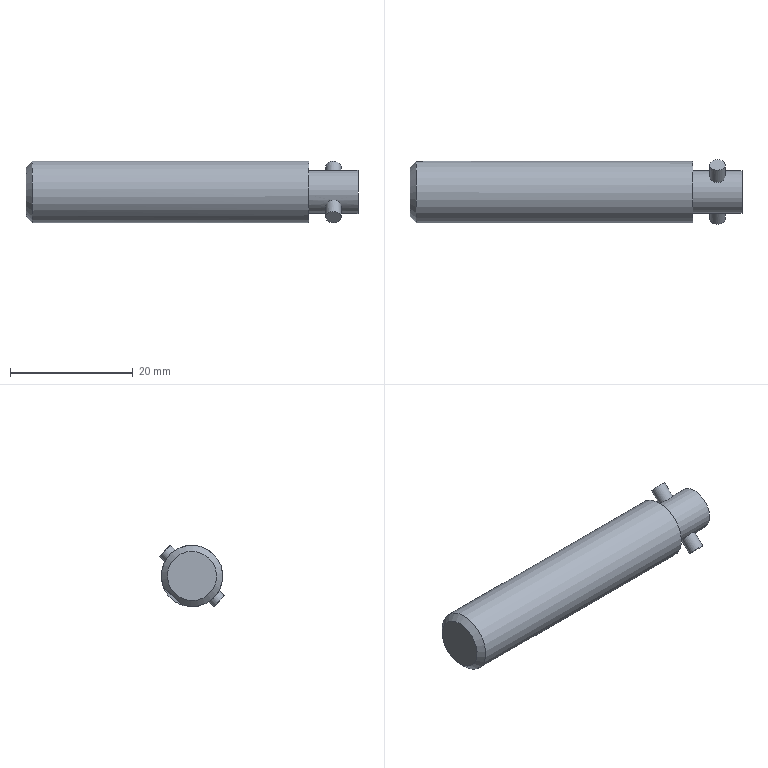Component | NX | 15B__27_2 | 1 solid | 12 faces | volume 3891 mm3 | plane 7 | cylinder 4 | cone 1 | commonest cylinder face diameters 2.5 x2 7 x1 10 x1